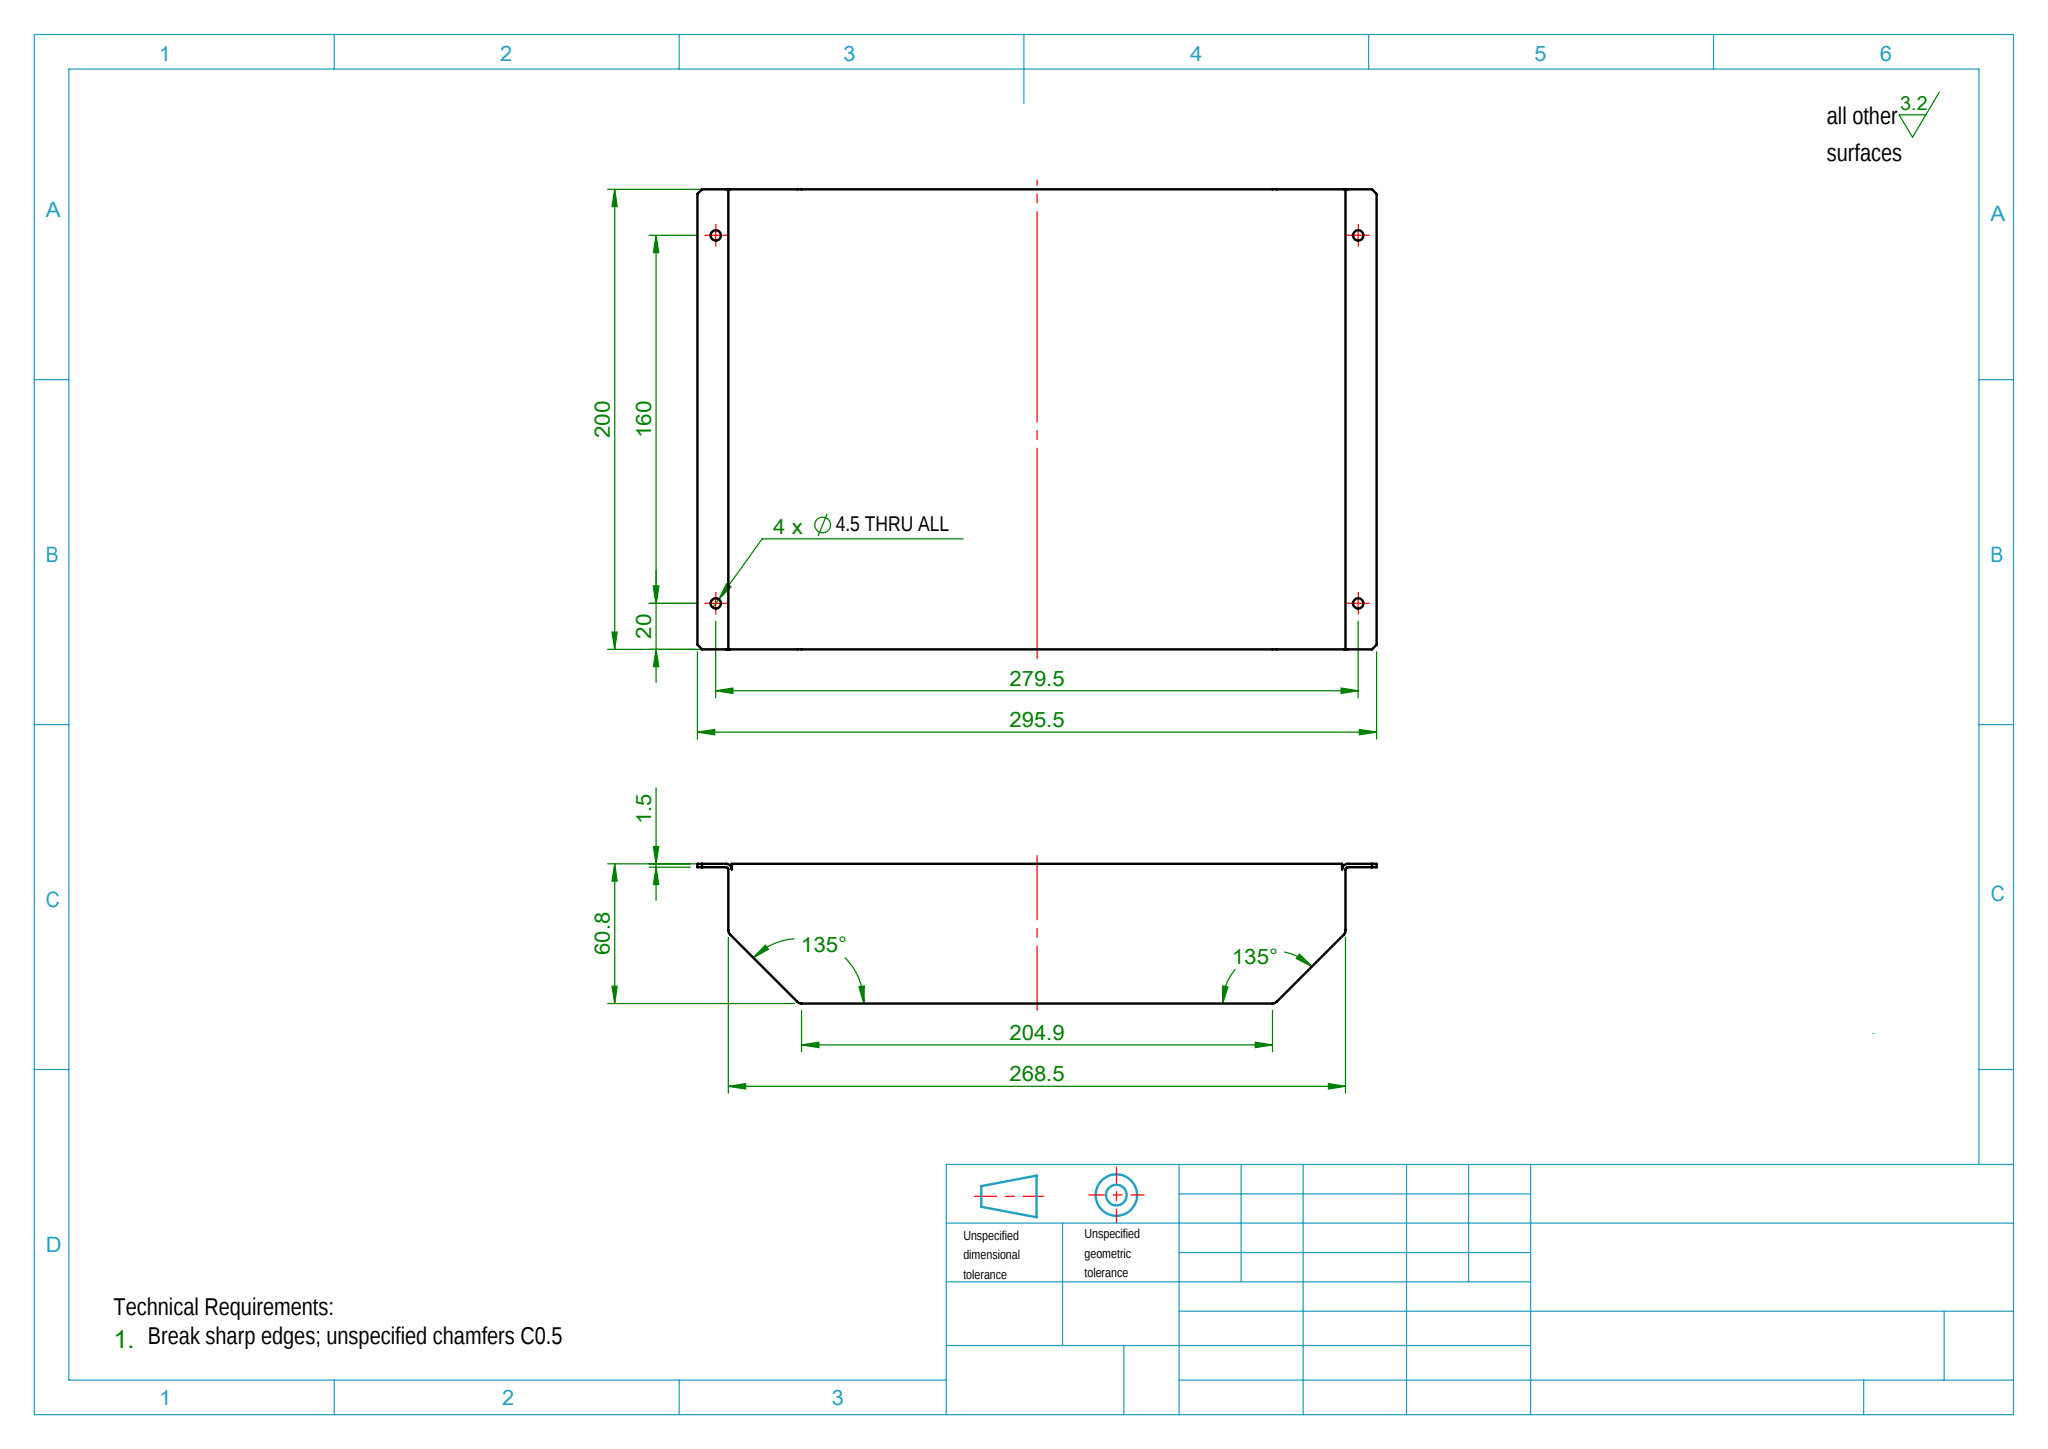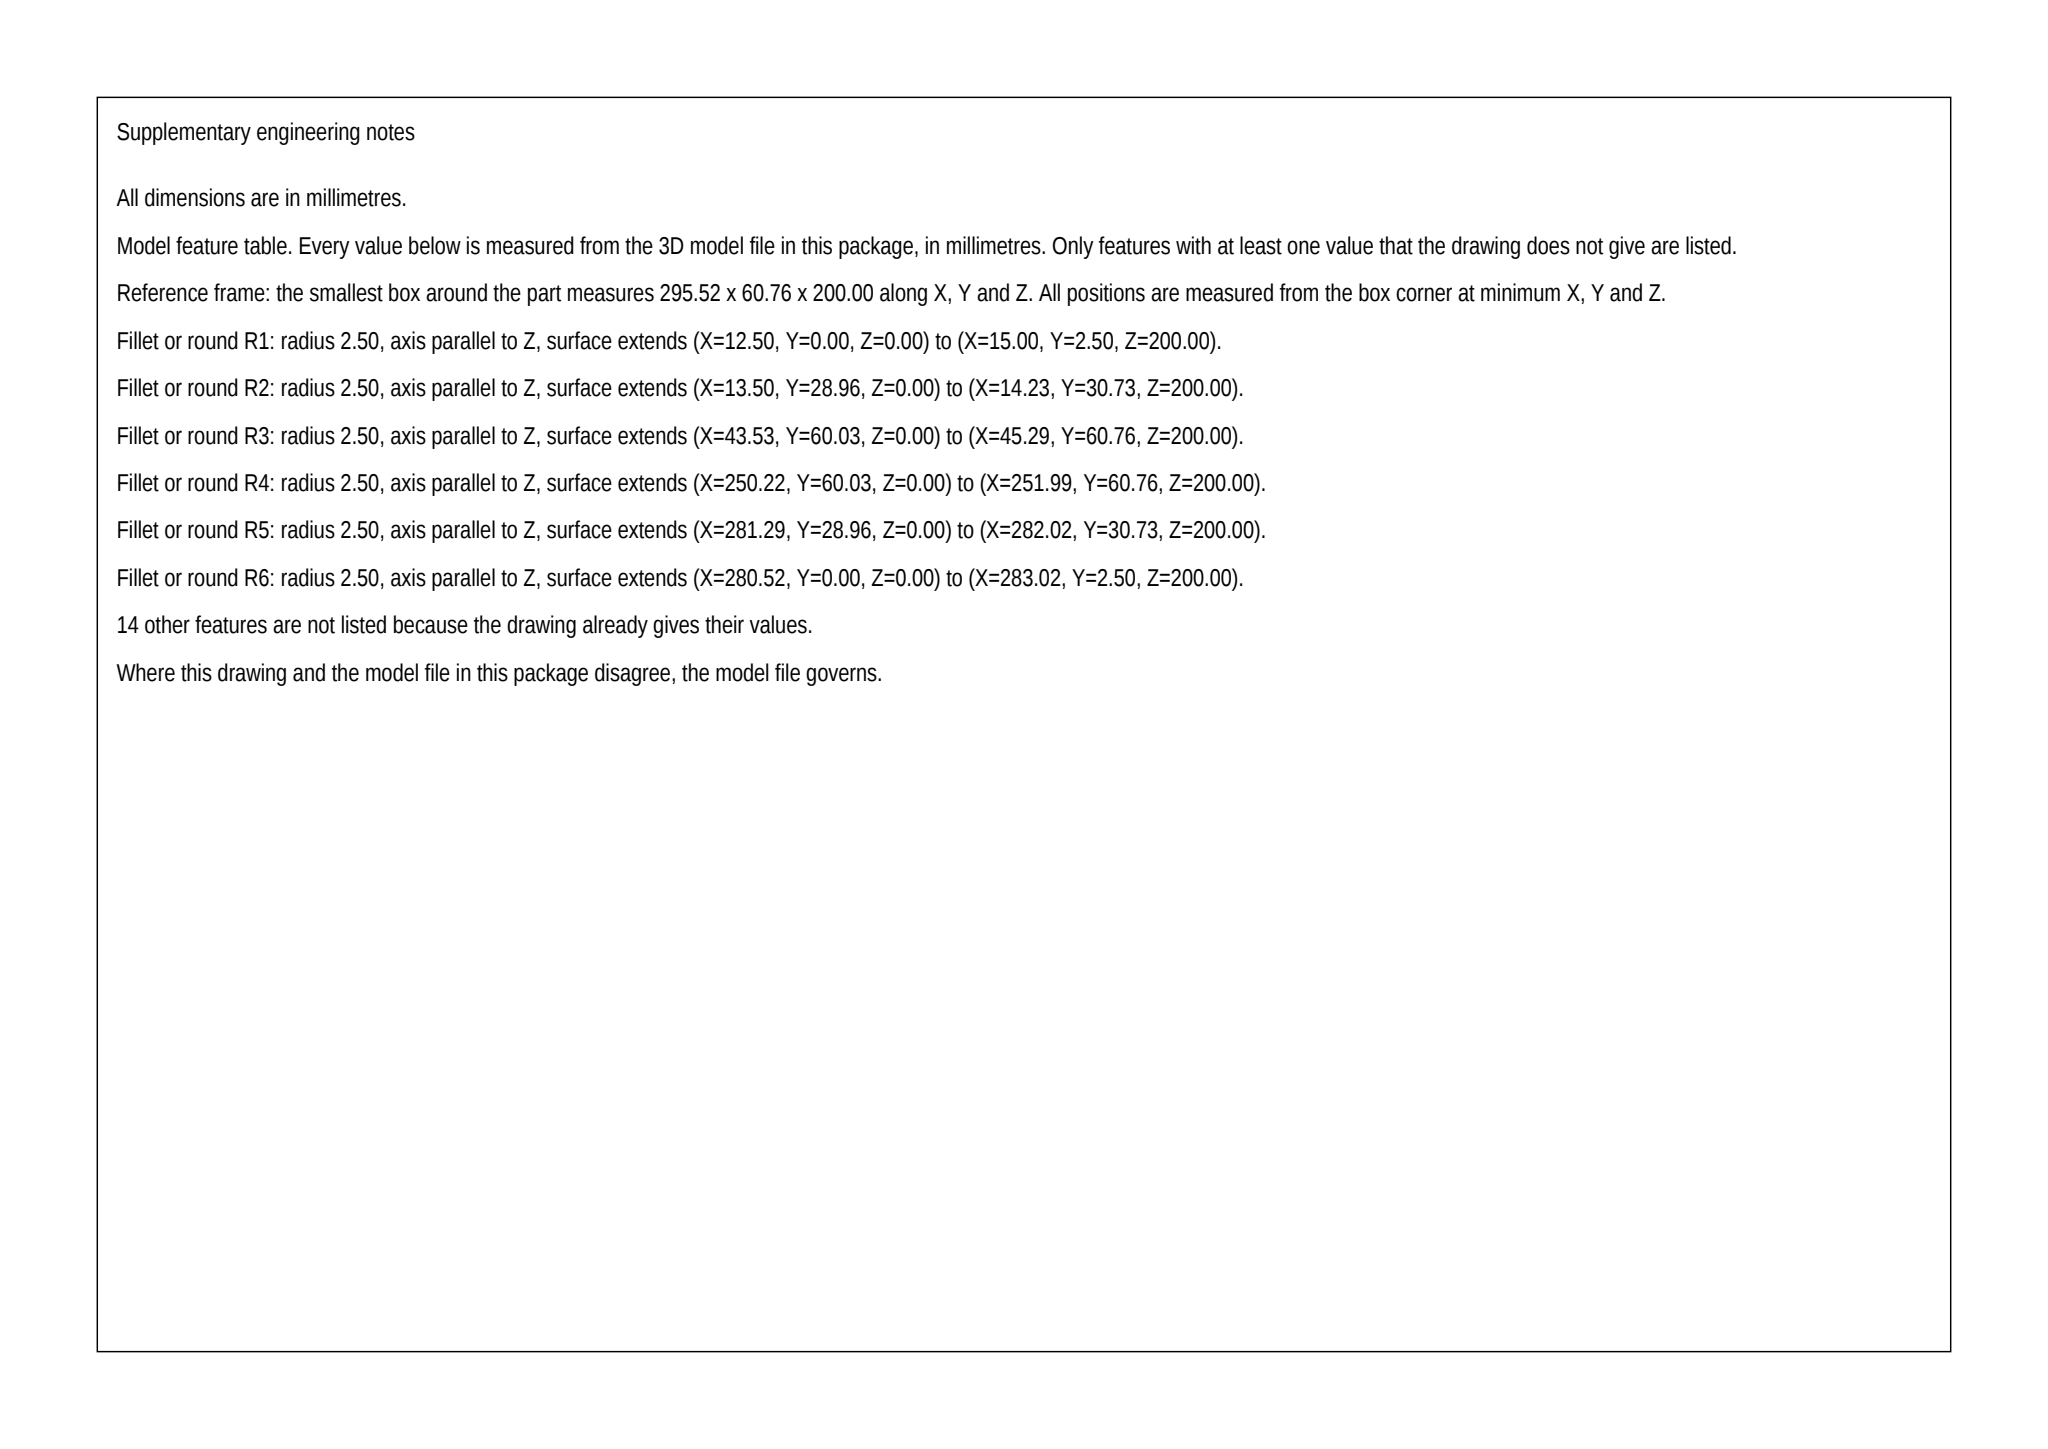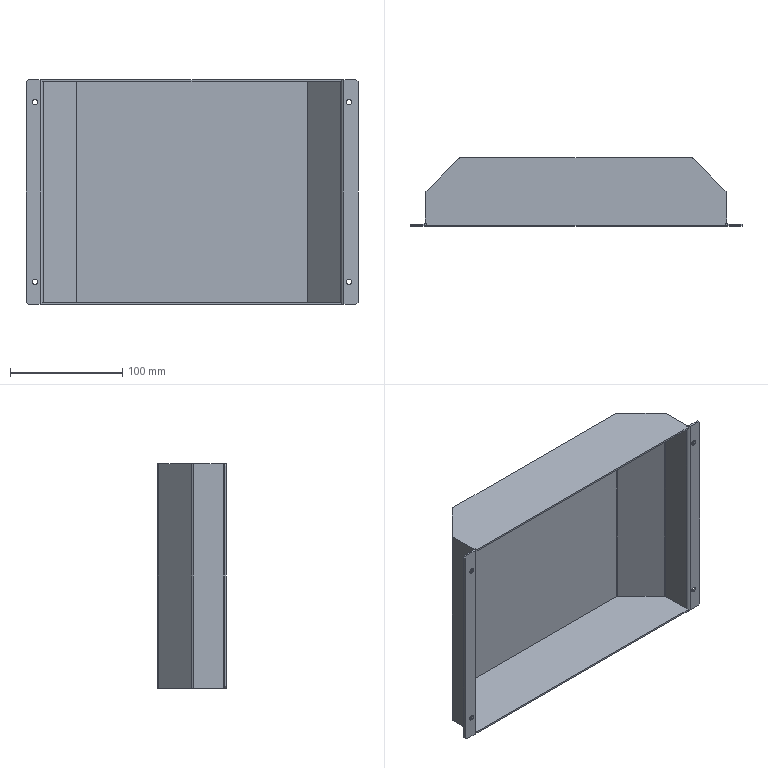Part | SolidWorks | mm | 1 solid | 58 faces | box 295.52 x 60.76 x 200 mm | volume 157430 mm3 | plane 38 | cylinder 20 | commonest cylinder face diameters 4.5 x8 2 x6 5 x6